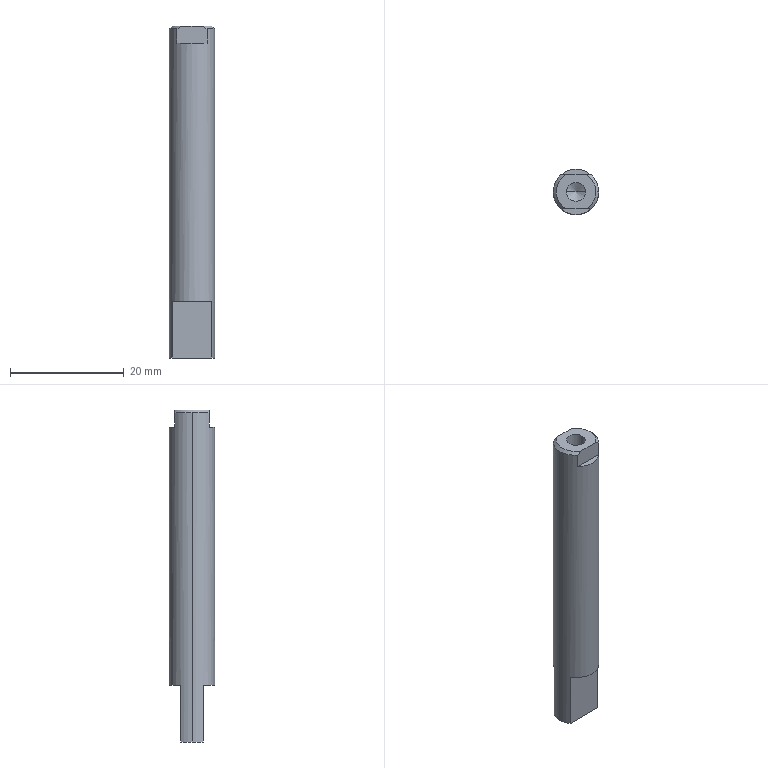Component | SolidWorks | 002MaterialPickingModuleA-1_004SidePlugModule-1_J-015-10 | 1 solid | 19 faces | box 8 x 8 x 58.4 mm | volume 2626 mm3 | plane 10 | cone 5 | cylinder 4 | commonest cylinder face diameters 3.3 x2 8 x2 | material 45
STEP:
#1=CARTESIAN_POINT('',(9.796,11.654,18.218));
#2=VERTEX_POINT('',#1);
#3=CARTESIAN_POINT('',(9.729,11.772,18.218));
#4=VERTEX_POINT('',#3);
#5=CARTESIAN_POINT('',(9.658,11.654,18.218));
#6=DIRECTION('',(0.,-0.,1.));
#7=DIRECTION('',(1.,0.,0.));
#8=AXIS2_PLACEMENT_3D('',#5,#6,#7);
#9=CIRCLE('',#8,0.1378);
#10=EDGE_CURVE('',#2,#4,#9,.T.);
#11=ORIENTED_EDGE('',*,*,#10,.F.);
#12=CARTESIAN_POINT('',(9.816,11.654,18.198));
#13=VERTEX_POINT('',#12);
#14=CARTESIAN_POINT('',(9.816,11.654,18.198));
#15=DIRECTION('',(0.7071,-0.,-0.7071));
#16=VECTOR('',#15,39.37);
#17=LINE('',#14,#16);
#18=EDGE_CURVE('',#2,#13,#17,.T.);
#19=ORIENTED_EDGE('',*,*,#18,.T.);
#20=CARTESIAN_POINT('',(9.763,11.772,18.198));
#21=VERTEX_POINT('',#20);
#22=CARTESIAN_POINT('',(9.658,11.654,18.198));
#23=DIRECTION('',(-0.,0.,-1.));
#24=DIRECTION('',(1.,0.,0.));
#25=AXIS2_PLACEMENT_3D('',#22,#23,#24);
#26=CIRCLE('',#25,0.1575);
#27=EDGE_CURVE('',#21,#13,#26,.T.);
#28=ORIENTED_EDGE('',*,*,#27,.F.);
#29=CARTESIAN_POINT('',(9.729,11.772,18.218));
#30=CARTESIAN_POINT('',(9.741,11.772,18.212));
#31=CARTESIAN_POINT('',(9.752,11.772,18.205));
#32=CARTESIAN_POINT('',(9.763,11.772,18.198));
#33=B_SPLINE_CURVE_WITH_KNOTS('',3,(#29,#30,#31,#32),.UNSPECIFIED.,.F.,.F.,(4,4),(0.008855,0.009835),.UNSPECIFIED.);
#34=EDGE_CURVE('',#4,#21,#33,.T.);
#35=ORIENTED_EDGE('',*,*,#34,.F.);
#36=EDGE_LOOP('',(#11,#19,#28,#35));
#37=FACE_OUTER_BOUND('',#36,.T.);
#38=CARTESIAN_POINT('',(9.658,11.654,18.198));
#39=DIRECTION('',(-0.,0.,-1.));
#40=DIRECTION('',(1.,0.,0.));
#41=AXIS2_PLACEMENT_3D('',#38,#39,#40);
#42=CONICAL_SURFACE('',#41,0.1575,0.7854);
#43=ADVANCED_FACE('',(#37),#42,.T.);
#44=CARTESIAN_POINT('',(9.723,11.654,17.82));
#45=VERTEX_POINT('',#44);
#46=CARTESIAN_POINT('',(9.593,11.654,17.82));
#47=VERTEX_POINT('',#46);
#48=CARTESIAN_POINT('',(9.658,11.654,17.82));
#49=DIRECTION('',(0.,-0.,1.));
#50=DIRECTION('',(-1.,0.,0.));
#51=AXIS2_PLACEMENT_3D('',#48,#49,#50);
#52=CIRCLE('',#51,0.06496);
#53=EDGE_CURVE('',#45,#47,#52,.T.);
#54=ORIENTED_EDGE('',*,*,#53,.F.);
#55=CARTESIAN_POINT('',(9.723,11.654,18.218));
#56=VERTEX_POINT('',#55);
#57=CARTESIAN_POINT('',(9.723,11.654,18.218));
#58=DIRECTION('',(0.,-0.,1.));
#59=VECTOR('',#58,39.37);
#60=LINE('',#57,#59);
#61=EDGE_CURVE('',#45,#56,#60,.T.);
#62=ORIENTED_EDGE('',*,*,#61,.T.);
#63=CARTESIAN_POINT('',(9.593,11.654,18.218));
#64=VERTEX_POINT('',#63);
#65=CARTESIAN_POINT('',(9.658,11.654,18.218));
#66=DIRECTION('',(0.,-0.,1.));
#67=DIRECTION('',(-1.,0.,0.));
#68=AXIS2_PLACEMENT_3D('',#65,#66,#67);
#69=CIRCLE('',#68,0.06496);
#70=EDGE_CURVE('',#56,#64,#69,.T.);
#71=ORIENTED_EDGE('',*,*,#70,.T.);
#72=CARTESIAN_POINT('',(9.593,11.654,18.218));
#73=DIRECTION('',(0.,-0.,1.));
#74=VECTOR('',#73,39.37);
#75=LINE('',#72,#74);
#76=EDGE_CURVE('',#47,#64,#75,.T.);
#77=ORIENTED_EDGE('',*,*,#76,.F.);
#78=EDGE_LOOP('',(#54,#62,#71,#77));
#79=FACE_OUTER_BOUND('',#78,.T.);
#80=CARTESIAN_POINT('',(9.658,11.654,18.218));
#81=DIRECTION('',(0.,-0.,1.));
#82=DIRECTION('',(-1.,0.,0.));
#83=AXIS2_PLACEMENT_3D('',#80,#81,#82);
#84=CYLINDRICAL_SURFACE('',#83,0.06496);
#85=ADVANCED_FACE('',(#79),#84,.F.);
#86=CARTESIAN_POINT('',(9.658,11.654,17.781));
#87=VERTEX_POINT('',#86);
#88=CARTESIAN_POINT('',(9.593,11.654,17.82));
#89=DIRECTION('',(-0.8572,0.,0.515));
#90=VECTOR('',#89,39.37);
#91=LINE('',#88,#90);
#92=EDGE_CURVE('',#87,#47,#91,.T.);
#93=ORIENTED_EDGE('',*,*,#92,.F.);
#94=CARTESIAN_POINT('',(9.723,11.654,17.82));
#95=DIRECTION('',(0.8572,-0.,0.515));
#96=VECTOR('',#95,39.37);
#97=LINE('',#94,#96);
#98=EDGE_CURVE('',#87,#45,#97,.T.);
#99=ORIENTED_EDGE('',*,*,#98,.T.);
#100=ORIENTED_EDGE('',*,*,#53,.T.);
#101=EDGE_LOOP('',(#93,#99,#100));
#102=FACE_OUTER_BOUND('',#101,.T.);
#103=CARTESIAN_POINT('',(9.658,11.654,17.82));
#104=DIRECTION('',(0.,-0.,1.));
#105=DIRECTION('',(-1.,0.,0.));
#106=AXIS2_PLACEMENT_3D('',#103,#104,#105);
#107=CONICAL_SURFACE('',#106,0.06496,1.03);
#108=ADVANCED_FACE('',(#102),#107,.F.);
#109=CARTESIAN_POINT('',(9.816,11.654,15.919));
#110=VERTEX_POINT('',#109);
#111=CARTESIAN_POINT('',(9.795,11.576,15.919));
#112=VERTEX_POINT('',#111);
#113=CARTESIAN_POINT('',(9.658,11.654,15.919));
#114=DIRECTION('',(-0.,0.,-1.));
#115=DIRECTION('',(1.,0.,0.));
#116=AXIS2_PLACEMENT_3D('',#113,#114,#115);
#117=CIRCLE('',#116,0.1575);
#118=EDGE_CURVE('',#110,#112,#117,.T.);
#119=ORIENTED_EDGE('',*,*,#118,.F.);
#120=CARTESIAN_POINT('',(9.816,11.654,15.919));
#121=DIRECTION('',(0.,-0.,1.));
#122=VECTOR('',#121,39.37);
#123=LINE('',#120,#122);
#124=EDGE_CURVE('',#110,#13,#123,.T.);
#125=ORIENTED_EDGE('',*,*,#124,.T.);
#126=CARTESIAN_POINT('',(9.763,11.536,18.198));
#127=VERTEX_POINT('',#126);
#128=CARTESIAN_POINT('',(9.658,11.654,18.198));
#129=DIRECTION('',(-0.,0.,-1.));
#130=DIRECTION('',(1.,0.,0.));
#131=AXIS2_PLACEMENT_3D('',#128,#129,#130);
#132=CIRCLE('',#131,0.1575);
#133=EDGE_CURVE('',#13,#127,#132,.T.);
#134=ORIENTED_EDGE('',*,*,#133,.T.);
#135=CARTESIAN_POINT('',(9.763,11.536,18.1));
#136=VERTEX_POINT('',#135);
#137=CARTESIAN_POINT('',(9.763,11.536,18.1));
#138=DIRECTION('',(0.,-0.,1.));
#139=VECTOR('',#138,39.37);
#140=LINE('',#137,#139);
#141=EDGE_CURVE('',#136,#127,#140,.T.);
#142=ORIENTED_EDGE('',*,*,#141,.F.);
#143=CARTESIAN_POINT('',(9.554,11.536,18.1));
#144=VERTEX_POINT('',#143);
#145=CARTESIAN_POINT('',(9.658,11.654,18.1));
#146=DIRECTION('',(0.,-0.,1.));
#147=DIRECTION('',(-1.,0.,0.));
#148=AXIS2_PLACEMENT_3D('',#145,#146,#147);
#149=CIRCLE('',#148,0.1575);
#150=EDGE_CURVE('',#144,#136,#149,.T.);
#151=ORIENTED_EDGE('',*,*,#150,.F.);
#152=CARTESIAN_POINT('',(9.554,11.536,18.198));
#153=VERTEX_POINT('',#152);
#154=CARTESIAN_POINT('',(9.554,11.536,18.1));
#155=DIRECTION('',(0.,-0.,1.));
#156=VECTOR('',#155,39.37);
#157=LINE('',#154,#156);
#158=EDGE_CURVE('',#144,#153,#157,.T.);
#159=ORIENTED_EDGE('',*,*,#158,.T.);
#160=CARTESIAN_POINT('',(9.501,11.654,18.198));
#161=VERTEX_POINT('',#160);
#162=CARTESIAN_POINT('',(9.658,11.654,18.198));
#163=DIRECTION('',(-0.,0.,-1.));
#164=DIRECTION('',(1.,0.,0.));
#165=AXIS2_PLACEMENT_3D('',#162,#163,#164);
#166=CIRCLE('',#165,0.1575);
#167=EDGE_CURVE('',#153,#161,#166,.T.);
#168=ORIENTED_EDGE('',*,*,#167,.T.);
#169=CARTESIAN_POINT('',(9.501,11.654,15.919));
#170=VERTEX_POINT('',#169);
#171=CARTESIAN_POINT('',(9.501,11.654,15.919));
#172=DIRECTION('',(0.,-0.,1.));
#173=VECTOR('',#172,39.37);
#174=LINE('',#171,#173);
#175=EDGE_CURVE('',#170,#161,#174,.T.);
#176=ORIENTED_EDGE('',*,*,#175,.F.);
#177=CARTESIAN_POINT('',(9.522,11.576,15.919));
#178=VERTEX_POINT('',#177);
#179=CARTESIAN_POINT('',(9.658,11.654,15.919));
#180=DIRECTION('',(-0.,0.,-1.));
#181=DIRECTION('',(1.,0.,0.));
#182=AXIS2_PLACEMENT_3D('',#179,#180,#181);
#183=CIRCLE('',#182,0.1575);
#184=EDGE_CURVE('',#178,#170,#183,.T.);
#185=ORIENTED_EDGE('',*,*,#184,.F.);
#186=CARTESIAN_POINT('',(9.522,11.576,16.312));
#187=VERTEX_POINT('',#186);
#188=CARTESIAN_POINT('',(9.522,11.576,16.312));
#189=DIRECTION('',(-0.,0.,-1.));
#190=VECTOR('',#189,39.37);
#191=LINE('',#188,#190);
#192=EDGE_CURVE('',#187,#178,#191,.T.);
#193=ORIENTED_EDGE('',*,*,#192,.F.);
#194=CARTESIAN_POINT('',(9.795,11.576,16.312));
#195=VERTEX_POINT('',#194);
#196=CARTESIAN_POINT('',(9.658,11.654,16.312));
#197=DIRECTION('',(-0.,0.,-1.));
#198=DIRECTION('',(1.,0.,0.));
#199=AXIS2_PLACEMENT_3D('',#196,#197,#198);
#200=CIRCLE('',#199,0.1575);
#201=EDGE_CURVE('',#195,#187,#200,.T.);
#202=ORIENTED_EDGE('',*,*,#201,.F.);
#203=CARTESIAN_POINT('',(9.795,11.576,16.312));
#204=DIRECTION('',(-0.,0.,-1.));
#205=VECTOR('',#204,39.37);
#206=LINE('',#203,#205);
#207=EDGE_CURVE('',#195,#112,#206,.T.);
#208=ORIENTED_EDGE('',*,*,#207,.T.);
#209=EDGE_LOOP('',(#119,#125,#134,#142,#151,#159,#168,#176,#185,#193,#202,#208));
#210=FACE_OUTER_BOUND('',#209,.T.);
#211=CARTESIAN_POINT('',(9.658,11.654,15.919));
#212=DIRECTION('',(0.,-0.,1.));
#213=DIRECTION('',(-1.,0.,0.));
#214=AXIS2_PLACEMENT_3D('',#211,#212,#213);
#215=CYLINDRICAL_SURFACE('',#214,0.1575);
#216=ADVANCED_FACE('',(#210),#215,.T.);
#217=CARTESIAN_POINT('',(9.554,11.772,18.198));
#218=VERTEX_POINT('',#217);
#219=CARTESIAN_POINT('',(9.587,11.772,18.218));
#220=VERTEX_POINT('',#219);
#221=CARTESIAN_POINT('',(9.554,11.772,18.198));
#222=CARTESIAN_POINT('',(9.565,11.772,18.205));
#223=CARTESIAN_POINT('',(9.576,11.772,18.212));
#224=CARTESIAN_POINT('',(9.587,11.772,18.218));
#225=B_SPLINE_CURVE_WITH_KNOTS('',3,(#221,#222,#223,#224),.UNSPECIFIED.,.F.,.F.,(4,4),(0.004095,0.005078),.UNSPECIFIED.);
#226=EDGE_CURVE('',#218,#220,#225,.T.);
#227=ORIENTED_EDGE('',*,*,#226,.F.);
#228=CARTESIAN_POINT('',(9.658,11.654,18.198));
#229=DIRECTION('',(-0.,0.,-1.));
#230=DIRECTION('',(1.,0.,0.));
#231=AXIS2_PLACEMENT_3D('',#228,#229,#230);
#232=CIRCLE('',#231,0.1575);
#233=EDGE_CURVE('',#161,#218,#232,.T.);
#234=ORIENTED_EDGE('',*,*,#233,.F.);
#235=ORIENTED_EDGE('',*,*,#167,.F.);
#236=CARTESIAN_POINT('',(9.587,11.536,18.218));
#237=VERTEX_POINT('',#236);
#238=CARTESIAN_POINT('',(9.587,11.536,18.218));
#239=CARTESIAN_POINT('',(9.576,11.536,18.212));
#240=CARTESIAN_POINT('',(9.565,11.536,18.205));
#241=CARTESIAN_POINT('',(9.554,11.536,18.198));
#242=B_SPLINE_CURVE_WITH_KNOTS('',3,(#238,#239,#240,#241),.UNSPECIFIED.,.F.,.F.,(4,4),(0.008855,0.009835),.UNSPECIFIED.);
#243=EDGE_CURVE('',#237,#153,#242,.T.);
#244=ORIENTED_EDGE('',*,*,#243,.F.);
#245=CARTESIAN_POINT('',(9.658,11.654,18.218));
#246=DIRECTION('',(0.,-0.,1.));
#247=DIRECTION('',(1.,0.,0.));
#248=AXIS2_PLACEMENT_3D('',#245,#246,#247);
#249=CIRCLE('',#248,0.1378);
#250=EDGE_CURVE('',#220,#237,#249,.T.);
#251=ORIENTED_EDGE('',*,*,#250,.F.);
#252=EDGE_LOOP('',(#227,#234,#235,#244,#251));
#253=FACE_OUTER_BOUND('',#252,.T.);
#254=CARTESIAN_POINT('',(9.658,11.654,18.198));
#255=DIRECTION('',(-0.,0.,-1.));
#256=DIRECTION('',(1.,0.,0.));
#257=AXIS2_PLACEMENT_3D('',#254,#255,#256);
#258=CONICAL_SURFACE('',#257,0.1575,0.7854);
#259=ADVANCED_FACE('',(#253),#258,.T.);
#260=ORIENTED_EDGE('',*,*,#124,.F.);
#261=CARTESIAN_POINT('',(9.795,11.733,15.919));
#262=VERTEX_POINT('',#261);
#263=CARTESIAN_POINT('',(9.658,11.654,15.919));
#264=DIRECTION('',(-0.,0.,-1.));
#265=DIRECTION('',(1.,0.,0.));
#266=AXIS2_PLACEMENT_3D('',#263,#264,#265);
#267=CIRCLE('',#266,0.1575);
#268=EDGE_CURVE('',#262,#110,#267,.T.);
#269=ORIENTED_EDGE('',*,*,#268,.F.);
#270=CARTESIAN_POINT('',(9.795,11.733,16.312));
#271=VERTEX_POINT('',#270);
#272=CARTESIAN_POINT('',(9.795,11.733,16.312));
#273=DIRECTION('',(-0.,0.,-1.));
#274=VECTOR('',#273,39.37);
#275=LINE('',#272,#274);
#276=EDGE_CURVE('',#271,#262,#275,.T.);
#277=ORIENTED_EDGE('',*,*,#276,.F.);
#278=CARTESIAN_POINT('',(9.522,11.733,16.312));
#279=VERTEX_POINT('',#278);
#280=CARTESIAN_POINT('',(9.658,11.654,16.312));
#281=DIRECTION('',(-0.,0.,-1.));
#282=DIRECTION('',(1.,0.,0.));
#283=AXIS2_PLACEMENT_3D('',#280,#281,#282);
#284=CIRCLE('',#283,0.1575);
#285=EDGE_CURVE('',#279,#271,#284,.T.);
#286=ORIENTED_EDGE('',*,*,#285,.F.);
#287=CARTESIAN_POINT('',(9.522,11.733,15.919));
#288=VERTEX_POINT('',#287);
#289=CARTESIAN_POINT('',(9.522,11.733,16.312));
#290=DIRECTION('',(-0.,0.,-1.));
#291=VECTOR('',#290,39.37);
#292=LINE('',#289,#291);
#293=EDGE_CURVE('',#279,#288,#292,.T.);
#294=ORIENTED_EDGE('',*,*,#293,.T.);
#295=CARTESIAN_POINT('',(9.658,11.654,15.919));
#296=DIRECTION('',(-0.,0.,-1.));
#297=DIRECTION('',(1.,0.,0.));
#298=AXIS2_PLACEMENT_3D('',#295,#296,#297);
#299=CIRCLE('',#298,0.1575);
#300=EDGE_CURVE('',#170,#288,#299,.T.);
#301=ORIENTED_EDGE('',*,*,#300,.F.);
#302=ORIENTED_EDGE('',*,*,#175,.T.);
#303=ORIENTED_EDGE('',*,*,#233,.T.);
#304=CARTESIAN_POINT('',(9.554,11.772,18.1));
#305=VERTEX_POINT('',#304);
#306=CARTESIAN_POINT('',(9.554,11.772,18.1));
#307=DIRECTION('',(0.,-0.,1.));
#308=VECTOR('',#307,39.37);
#309=LINE('',#306,#308);
#310=EDGE_CURVE('',#305,#218,#309,.T.);
#311=ORIENTED_EDGE('',*,*,#310,.F.);
#312=CARTESIAN_POINT('',(9.763,11.772,18.1));
#313=VERTEX_POINT('',#312);
#314=CARTESIAN_POINT('',(9.658,11.654,18.1));
#315=DIRECTION('',(0.,-0.,1.));
#316=DIRECTION('',(-1.,0.,0.));
#317=AXIS2_PLACEMENT_3D('',#314,#315,#316);
#318=CIRCLE('',#317,0.1575);
#319=EDGE_CURVE('',#313,#305,#318,.T.);
#320=ORIENTED_EDGE('',*,*,#319,.F.);
#321=CARTESIAN_POINT('',(9.763,11.772,18.1));
#322=DIRECTION('',(0.,-0.,1.));
#323=VECTOR('',#322,39.37);
#324=LINE('',#321,#323);
#325=EDGE_CURVE('',#313,#21,#324,.T.);
#326=ORIENTED_EDGE('',*,*,#325,.T.);
#327=ORIENTED_EDGE('',*,*,#27,.T.);
#328=EDGE_LOOP('',(#260,#269,#277,#286,#294,#301,#302,#303,#311,#320,#326,#327));
#329=FACE_OUTER_BOUND('',#328,.T.);
#330=CARTESIAN_POINT('',(9.658,11.654,15.919));
#331=DIRECTION('',(0.,-0.,1.));
#332=DIRECTION('',(-1.,0.,0.));
#333=AXIS2_PLACEMENT_3D('',#330,#331,#332);
#334=CYLINDRICAL_SURFACE('',#333,0.1575);
#335=ADVANCED_FACE('',(#329),#334,.T.);
#336=CARTESIAN_POINT('',(9.795,11.733,15.919));
#337=DIRECTION('',(-1.,0.,0.));
#338=VECTOR('',#337,39.37);
#339=LINE('',#336,#338);
#340=EDGE_CURVE('',#262,#288,#339,.T.);
#341=ORIENTED_EDGE('',*,*,#340,.F.);
#342=ORIENTED_EDGE('',*,*,#268,.T.);
#343=ORIENTED_EDGE('',*,*,#118,.T.);
#344=CARTESIAN_POINT('',(9.795,11.576,15.919));
#345=DIRECTION('',(1.,-0.,-0.));
#346=VECTOR('',#345,39.37);
#347=LINE('',#344,#346);
#348=EDGE_CURVE('',#178,#112,#347,.T.);
#349=ORIENTED_EDGE('',*,*,#348,.F.);
#350=ORIENTED_EDGE('',*,*,#184,.T.);
#351=ORIENTED_EDGE('',*,*,#300,.T.);
#352=EDGE_LOOP('',(#341,#342,#343,#349,#350,#351));
#353=FACE_OUTER_BOUND('',#352,.T.);
#354=CARTESIAN_POINT('',(9.658,11.654,15.919));
#355=DIRECTION('',(-0.,0.,-1.));
#356=DIRECTION('',(1.,-0.,-0.));
#357=AXIS2_PLACEMENT_3D('',#354,#355,#356);
#358=PLANE('',#357);
#359=ADVANCED_FACE('',(#353),#358,.T.);
#360=CARTESIAN_POINT('',(9.729,11.536,18.218));
#361=VERTEX_POINT('',#360);
#362=CARTESIAN_POINT('',(9.658,11.654,18.218));
#363=DIRECTION('',(0.,-0.,1.));
#364=DIRECTION('',(1.,0.,0.));
#365=AXIS2_PLACEMENT_3D('',#362,#363,#364);
#366=CIRCLE('',#365,0.1378);
#367=EDGE_CURVE('',#361,#2,#366,.T.);
#368=ORIENTED_EDGE('',*,*,#367,.T.);
#369=ORIENTED_EDGE('',*,*,#10,.T.);
#370=CARTESIAN_POINT('',(9.554,11.772,18.218));
#371=DIRECTION('',(1.,-0.,-0.));
#372=VECTOR('',#371,39.37);
#373=LINE('',#370,#372);
#374=EDGE_CURVE('',#220,#4,#373,.T.);
#375=ORIENTED_EDGE('',*,*,#374,.F.);
#376=ORIENTED_EDGE('',*,*,#250,.T.);
#377=CARTESIAN_POINT('',(9.554,11.536,18.218));
#378=DIRECTION('',(-1.,0.,0.));
#379=VECTOR('',#378,39.37);
#380=LINE('',#377,#379);
#381=EDGE_CURVE('',#361,#237,#380,.T.);
#382=ORIENTED_EDGE('',*,*,#381,.F.);
#383=EDGE_LOOP('',(#368,#369,#375,#376,#382));
#384=FACE_OUTER_BOUND('',#383,.T.);
#385=CARTESIAN_POINT('',(9.658,11.654,18.218));
#386=DIRECTION('',(0.,-0.,1.));
#387=DIRECTION('',(-1.,0.,0.));
#388=AXIS2_PLACEMENT_3D('',#385,#386,#387);
#389=CIRCLE('',#388,0.06496);
#390=EDGE_CURVE('',#64,#56,#389,.T.);
#391=ORIENTED_EDGE('',*,*,#390,.F.);
#392=ORIENTED_EDGE('',*,*,#70,.F.);
#393=EDGE_LOOP('',(#391,#392));
#394=FACE_BOUND('',#393,.T.);
#395=CARTESIAN_POINT('',(9.658,11.654,18.218));
#396=DIRECTION('',(-0.,0.,-1.));
#397=DIRECTION('',(1.,-0.,-0.));
#398=AXIS2_PLACEMENT_3D('',#395,#396,#397);
#399=PLANE('',#398);
#400=ADVANCED_FACE('',(#384,#394),#399,.F.);
#401=ORIENTED_EDGE('',*,*,#348,.T.);
#402=ORIENTED_EDGE('',*,*,#207,.F.);
#403=CARTESIAN_POINT('',(9.795,11.576,16.312));
#404=DIRECTION('',(1.,-0.,-0.));
#405=VECTOR('',#404,39.37);
#406=LINE('',#403,#405);
#407=EDGE_CURVE('',#187,#195,#406,.T.);
#408=ORIENTED_EDGE('',*,*,#407,.F.);
#409=ORIENTED_EDGE('',*,*,#192,.T.);
#410=EDGE_LOOP('',(#401,#402,#408,#409));
#411=FACE_OUTER_BOUND('',#410,.T.);
#412=CARTESIAN_POINT('',(9.795,11.576,16.312));
#413=DIRECTION('',(0.,1.,0.));
#414=DIRECTION('',(0.,-0.,1.));
#415=AXIS2_PLACEMENT_3D('',#412,#413,#414);
#416=PLANE('',#415);
#417=ADVANCED_FACE('',(#411),#416,.F.);
#418=ORIENTED_EDGE('',*,*,#201,.T.);
#419=ORIENTED_EDGE('',*,*,#407,.T.);
#420=EDGE_LOOP('',(#418,#419));
#421=FACE_OUTER_BOUND('',#420,.T.);
#422=CARTESIAN_POINT('',(9.658,11.654,16.312));
#423=DIRECTION('',(-0.,0.,-1.));
#424=DIRECTION('',(1.,-0.,-0.));
#425=AXIS2_PLACEMENT_3D('',#422,#423,#424);
#426=PLANE('',#425);
#427=ADVANCED_FACE('',(#421),#426,.T.);
#428=ORIENTED_EDGE('',*,*,#340,.T.);
#429=ORIENTED_EDGE('',*,*,#293,.F.);
#430=CARTESIAN_POINT('',(9.795,11.733,16.312));
#431=DIRECTION('',(-1.,0.,0.));
#432=VECTOR('',#431,39.37);
#433=LINE('',#430,#432);
#434=EDGE_CURVE('',#271,#279,#433,.T.);
#435=ORIENTED_EDGE('',*,*,#434,.F.);
#436=ORIENTED_EDGE('',*,*,#276,.T.);
#437=EDGE_LOOP('',(#428,#429,#435,#436));
#438=FACE_OUTER_BOUND('',#437,.T.);
#439=CARTESIAN_POINT('',(9.795,11.733,16.312));
#440=DIRECTION('',(-0.,-1.,-0.));
#441=DIRECTION('',(-0.,0.,-1.));
#442=AXIS2_PLACEMENT_3D('',#439,#440,#441);
#443=PLANE('',#442);
#444=ADVANCED_FACE('',(#438),#443,.F.);
#445=ORIENTED_EDGE('',*,*,#285,.T.);
#446=ORIENTED_EDGE('',*,*,#434,.T.);
#447=EDGE_LOOP('',(#445,#446));
#448=FACE_OUTER_BOUND('',#447,.T.);
#449=CARTESIAN_POINT('',(9.658,11.654,16.312));
#450=DIRECTION('',(-0.,0.,-1.));
#451=DIRECTION('',(1.,-0.,-0.));
#452=AXIS2_PLACEMENT_3D('',#449,#450,#451);
#453=PLANE('',#452);
#454=ADVANCED_FACE('',(#448),#453,.T.);
#455=ORIENTED_EDGE('',*,*,#98,.F.);
#456=ORIENTED_EDGE('',*,*,#92,.T.);
#457=CARTESIAN_POINT('',(9.658,11.654,17.82));
#458=DIRECTION('',(0.,-0.,1.));
#459=DIRECTION('',(-1.,0.,0.));
#460=AXIS2_PLACEMENT_3D('',#457,#458,#459);
#461=CIRCLE('',#460,0.06496);
#462=EDGE_CURVE('',#47,#45,#461,.T.);
#463=ORIENTED_EDGE('',*,*,#462,.T.);
#464=EDGE_LOOP('',(#455,#456,#463));
#465=FACE_OUTER_BOUND('',#464,.T.);
#466=CARTESIAN_POINT('',(9.658,11.654,17.82));
#467=DIRECTION('',(0.,-0.,1.));
#468=DIRECTION('',(-1.,0.,0.));
#469=AXIS2_PLACEMENT_3D('',#466,#467,#468);
#470=CONICAL_SURFACE('',#469,0.06496,1.03);
#471=ADVANCED_FACE('',(#465),#470,.F.);
#472=ORIENTED_EDGE('',*,*,#61,.F.);
#473=ORIENTED_EDGE('',*,*,#462,.F.);
#474=ORIENTED_EDGE('',*,*,#76,.T.);
#475=ORIENTED_EDGE('',*,*,#390,.T.);
#476=EDGE_LOOP('',(#472,#473,#474,#475));
#477=FACE_OUTER_BOUND('',#476,.T.);
#478=CARTESIAN_POINT('',(9.658,11.654,18.218));
#479=DIRECTION('',(0.,-0.,1.));
#480=DIRECTION('',(-1.,0.,0.));
#481=AXIS2_PLACEMENT_3D('',#478,#479,#480);
#482=CYLINDRICAL_SURFACE('',#481,0.06496);
#483=ADVANCED_FACE('',(#477),#482,.F.);
#484=ORIENTED_EDGE('',*,*,#18,.F.);
#485=ORIENTED_EDGE('',*,*,#367,.F.);
#486=CARTESIAN_POINT('',(9.763,11.536,18.198));
#487=CARTESIAN_POINT('',(9.752,11.536,18.205));
#488=CARTESIAN_POINT('',(9.741,11.536,18.212));
#489=CARTESIAN_POINT('',(9.729,11.536,18.218));
#490=B_SPLINE_CURVE_WITH_KNOTS('',3,(#486,#487,#488,#489),.UNSPECIFIED.,.F.,.F.,(4,4),(0.004095,0.005078),.UNSPECIFIED.);
#491=EDGE_CURVE('',#127,#361,#490,.T.);
#492=ORIENTED_EDGE('',*,*,#491,.F.);
#493=ORIENTED_EDGE('',*,*,#133,.F.);
#494=EDGE_LOOP('',(#484,#485,#492,#493));
#495=FACE_OUTER_BOUND('',#494,.T.);
#496=CARTESIAN_POINT('',(9.658,11.654,18.198));
#497=DIRECTION('',(-0.,0.,-1.));
#498=DIRECTION('',(1.,0.,0.));
#499=AXIS2_PLACEMENT_3D('',#496,#497,#498);
#500=CONICAL_SURFACE('',#499,0.1575,0.7854);
#501=ADVANCED_FACE('',(#495),#500,.T.);
#502=ORIENTED_EDGE('',*,*,#491,.T.);
#503=ORIENTED_EDGE('',*,*,#381,.T.);
#504=ORIENTED_EDGE('',*,*,#243,.T.);
#505=ORIENTED_EDGE('',*,*,#158,.F.);
#506=CARTESIAN_POINT('',(9.554,11.536,18.1));
#507=DIRECTION('',(-1.,0.,0.));
#508=VECTOR('',#507,39.37);
#509=LINE('',#506,#508);
#510=EDGE_CURVE('',#136,#144,#509,.T.);
#511=ORIENTED_EDGE('',*,*,#510,.F.);
#512=ORIENTED_EDGE('',*,*,#141,.T.);
#513=EDGE_LOOP('',(#502,#503,#504,#505,#511,#512));
#514=FACE_OUTER_BOUND('',#513,.T.);
#515=CARTESIAN_POINT('',(9.554,11.536,18.1));
#516=DIRECTION('',(0.,1.,0.));
#517=DIRECTION('',(0.,-0.,1.));
#518=AXIS2_PLACEMENT_3D('',#515,#516,#517);
#519=PLANE('',#518);
#520=ADVANCED_FACE('',(#514),#519,.F.);
#521=ORIENTED_EDGE('',*,*,#150,.T.);
#522=ORIENTED_EDGE('',*,*,#510,.T.);
#523=EDGE_LOOP('',(#521,#522));
#524=FACE_OUTER_BOUND('',#523,.T.);
#525=CARTESIAN_POINT('',(9.658,11.654,18.1));
#526=DIRECTION('',(0.,-0.,1.));
#527=DIRECTION('',(-1.,0.,0.));
#528=AXIS2_PLACEMENT_3D('',#525,#526,#527);
#529=PLANE('',#528);
#530=ADVANCED_FACE('',(#524),#529,.T.);
#531=ORIENTED_EDGE('',*,*,#226,.T.);
#532=ORIENTED_EDGE('',*,*,#374,.T.);
#533=ORIENTED_EDGE('',*,*,#34,.T.);
#534=ORIENTED_EDGE('',*,*,#325,.F.);
#535=CARTESIAN_POINT('',(9.554,11.772,18.1));
#536=DIRECTION('',(1.,-0.,-0.));
#537=VECTOR('',#536,39.37);
#538=LINE('',#535,#537);
#539=EDGE_CURVE('',#305,#313,#538,.T.);
#540=ORIENTED_EDGE('',*,*,#539,.F.);
#541=ORIENTED_EDGE('',*,*,#310,.T.);
#542=EDGE_LOOP('',(#531,#532,#533,#534,#540,#541));
#543=FACE_OUTER_BOUND('',#542,.T.);
#544=CARTESIAN_POINT('',(9.554,11.772,18.1));
#545=DIRECTION('',(-0.,-1.,-0.));
#546=DIRECTION('',(-0.,0.,-1.));
#547=AXIS2_PLACEMENT_3D('',#544,#545,#546);
#548=PLANE('',#547);
#549=ADVANCED_FACE('',(#543),#548,.F.);
#550=ORIENTED_EDGE('',*,*,#319,.T.);
#551=ORIENTED_EDGE('',*,*,#539,.T.);
#552=EDGE_LOOP('',(#550,#551));
#553=FACE_OUTER_BOUND('',#552,.T.);
#554=CARTESIAN_POINT('',(9.658,11.654,18.1));
#555=DIRECTION('',(0.,-0.,1.));
#556=DIRECTION('',(-1.,0.,0.));
#557=AXIS2_PLACEMENT_3D('',#554,#555,#556);
#558=PLANE('',#557);
#559=ADVANCED_FACE('',(#553),#558,.T.);
#560=CLOSED_SHELL('',(#43,#85,#108,#216,#259,#335,#359,#400,#417,#427,#444,#454,#471,#483,#501,#520,#530,#549,#559));
#561=MANIFOLD_SOLID_BREP('',#560);
#562=CARTESIAN_POINT('',(0.,0.,0.));
#563=DIRECTION('',(0.,0.,1.));
#564=DIRECTION('',(1.,0.,0.));
#565=AXIS2_PLACEMENT_3D('',#562,#563,#564);
#566=(LENGTH_UNIT()NAMED_UNIT(*)SI_UNIT($,.METRE.));
#567=LENGTH_MEASURE_WITH_UNIT(LENGTH_MEASURE(0.0254),#566);
#568=DIMENSIONAL_EXPONENTS(1.,0.,0.,0.,0.,0.,0.);
#569=(CONVERSION_BASED_UNIT('',#567)LENGTH_UNIT()NAMED_UNIT(#568));
#570=UNCERTAINTY_MEASURE_WITH_UNIT(LENGTH_MEASURE(0.00001),#569,'','');
#571=(NAMED_UNIT(*)PLANE_ANGLE_UNIT()SI_UNIT($,.RADIAN.));
#572=(NAMED_UNIT(*)SI_UNIT($,.STERADIAN.)SOLID_ANGLE_UNIT());
#573=(GEOMETRIC_REPRESENTATION_CONTEXT(3)GLOBAL_UNCERTAINTY_ASSIGNED_CONTEXT((#570))GLOBAL_UNIT_ASSIGNED_CONTEXT((#569,#571,#572))REPRESENTATION_CONTEXT('',''));
#574=ADVANCED_BREP_SHAPE_REPRESENTATION('',(#561,#565),#573);
#575=COLOUR_RGB('',0.7922,0.8196,0.9333);
#576=FILL_AREA_STYLE_COLOUR('',#575);
#577=FILL_AREA_STYLE('',(#576));
#578=SURFACE_STYLE_FILL_AREA(#577);
#579=SURFACE_SIDE_STYLE('',(#578));
#580=SURFACE_STYLE_USAGE(.BOTH.,#579);
#581=PRESENTATION_STYLE_ASSIGNMENT((#580));
#582=STYLED_ITEM('',(#581),#561);
#583=(LENGTH_UNIT()NAMED_UNIT(*)SI_UNIT($,.METRE.));
#584=LENGTH_MEASURE_WITH_UNIT(LENGTH_MEASURE(0.0254),#583);
#585=DIMENSIONAL_EXPONENTS(1.,0.,0.,0.,0.,0.,0.);
#586=(CONVERSION_BASED_UNIT('',#584)LENGTH_UNIT()NAMED_UNIT(#585));
#587=UNCERTAINTY_MEASURE_WITH_UNIT(LENGTH_MEASURE(0.00001),#586,'','');
#588=(NAMED_UNIT(*)PLANE_ANGLE_UNIT()SI_UNIT($,.RADIAN.));
#589=(NAMED_UNIT(*)SI_UNIT($,.STERADIAN.)SOLID_ANGLE_UNIT());
#590=(GEOMETRIC_REPRESENTATION_CONTEXT(3)GLOBAL_UNCERTAINTY_ASSIGNED_CONTEXT((#587))GLOBAL_UNIT_ASSIGNED_CONTEXT((#586,#588,#589))REPRESENTATION_CONTEXT('',''));
#591=MECHANICAL_DESIGN_GEOMETRIC_PRESENTATION_REPRESENTATION('',(#582),#590);
#592=PRESENTATION_LAYER_ASSIGNMENT('','',(#582));